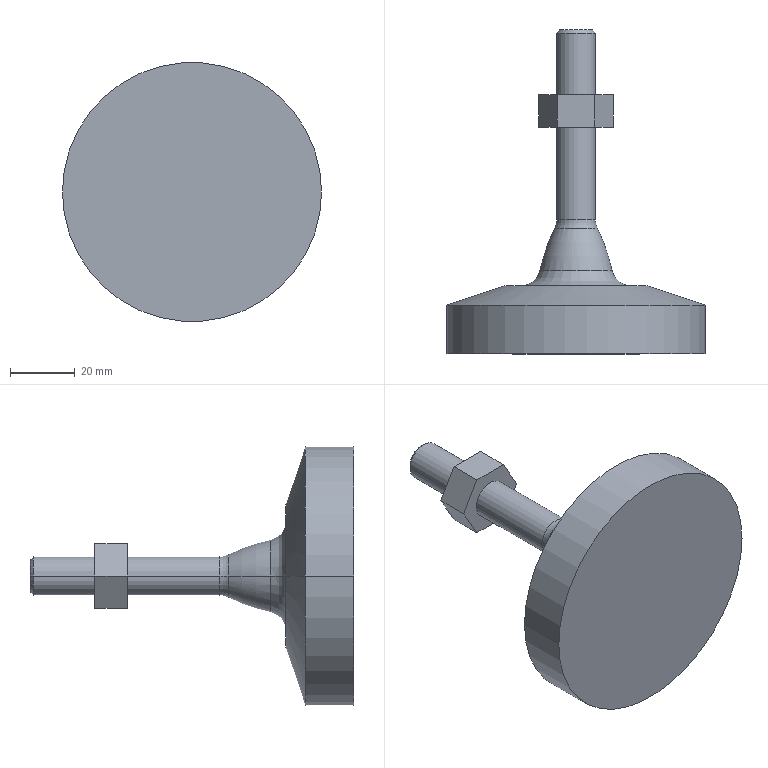Component | SolidWorks | FrameAssembly-1_FootCup-3 | 1 solid | 27 faces | box 80 x 100 x 80 mm | volume 109185 mm3 | plane 11 | torus 6 | cylinder 6 | cone 4 | commonest cylinder face diameters 12 x4 80 x2
build123d program:
from build123d import *

# Parameters (mm, degrees)
BOSS_EXTRUDE1_DEPTH = 10
FILLET1_R           = 6


with BuildPart() as part:
    # Sketch1 → Boss-Extrude1 (new body)
    with BuildSketch(Plane(origin=(0, 80, 0), x_dir=(1, 0, 0), z_dir=(0, 1, 0))):
        Polygon((-5.774, 10), (-11.547, 0), (-5.774, -10), (5.774, -10), (11.547, 0), (5.774, 10), align=None)
    extrude(amount=-BOSS_EXTRUDE1_DEPTH)

    # Sketch2 → Revolve1 (revolve)
    with BuildSketch(Plane(origin=(0, 0, 0), x_dir=(-1, 0, 0), z_dir=(0, 0, -1)), mode=Mode.PRIVATE) as revolve1_sk:
        with BuildLine():
            Line((-40, 0), (0, 0))
            Line((0, 0), (0, 70))
            Line((0, 70), (-6, 70))
            Line((-6, 70), (-6, 40))
            ThreePointArc((-6, 40), (-9.794, 30.751), (-12, 21))
            Line((-12, 21), (-22, 21))
            Line((-22, 21), (-40, 15))
            Line((-40, 15), (-40, 0))
        make_face()
    revolve(revolve1_sk.sketch.rotate(Axis((0, 0, 0), (0, 1, 0)), 180), axis=Axis((0, 0, 0), (0, 1, 0)))

    # Sketch3 → Revolve2 (revolve)
    with BuildSketch(Plane(origin=(0, 0, 0), x_dir=(-1, 0, 0), z_dir=(0, 0, -1)), mode=Mode.PRIVATE) as revolve2_sk:
        Polygon((-6, 80), (0, 80), (0, 100), (-5, 100), (-6, 99), align=None)
    revolve(revolve2_sk.sketch.rotate(Axis((0, 80, 0), (0, 1, 0)), 180), axis=Axis((0, 80, 0), (0, 1, 0)))

    # Fillet1
    fillet1_edges = [part.edges().sort_by_distance(p)[0] for p in [
        (6, 40, 0),
        (12, 21, 0),
    ]]
    fillet(fillet1_edges, radius=FILLET1_R)


solid = part.part

# Placed as in the assembly
solid = solid.moved(Location((-641.246, -528.627, -346.5), (0, 0, 0)))
STEP:
#1=COLOUR_RGB('',0.7922,0.8196,0.9333);
#2=FILL_AREA_STYLE_COLOUR('',#1);
#3=FILL_AREA_STYLE('',(#2));
#4=SURFACE_STYLE_FILL_AREA(#3);
#5=SURFACE_SIDE_STYLE('',(#4));
#6=SURFACE_STYLE_USAGE(.BOTH.,#5);
#7=PRESENTATION_STYLE_ASSIGNMENT((#6));
#8=CARTESIAN_POINT('',(-25.01,-19.182,-13.642));
#9=VERTEX_POINT('',#8);
#10=CARTESIAN_POINT('',(-25.482,-19.182,-13.642));
#11=VERTEX_POINT('',#10);
#12=CARTESIAN_POINT('',(-25.246,-19.182,-13.642));
#13=DIRECTION('',(0.,1.,0.));
#14=DIRECTION('',(-1.,0.,0.));
#15=AXIS2_PLACEMENT_3D('',#12,#13,#14);
#16=CIRCLE('',#15,0.2362);
#17=EDGE_CURVE('',#9,#11,#16,.T.);
#18=ORIENTED_EDGE('',*,*,#17,.F.);
#19=CARTESIAN_POINT('',(-24.986,-19.285,-13.642));
#20=VERTEX_POINT('',#19);
#21=CARTESIAN_POINT('',(-24.773,-19.182,-13.642));
#22=DIRECTION('',(-0.,0.,1.));
#23=DIRECTION('',(1.,0.,0.));
#24=AXIS2_PLACEMENT_3D('',#21,#22,#23);
#25=CIRCLE('',#24,0.2362);
#26=EDGE_CURVE('',#9,#20,#25,.T.);
#27=ORIENTED_EDGE('',*,*,#26,.T.);
#28=CARTESIAN_POINT('',(-25.506,-19.285,-13.642));
#29=VERTEX_POINT('',#28);
#30=CARTESIAN_POINT('',(-25.246,-19.285,-13.642));
#31=DIRECTION('',(-0.,-1.,0.));
#32=DIRECTION('',(1.,0.,0.));
#33=AXIS2_PLACEMENT_3D('',#30,#31,#32);
#34=CIRCLE('',#33,0.2598);
#35=EDGE_CURVE('',#29,#20,#34,.T.);
#36=ORIENTED_EDGE('',*,*,#35,.F.);
#37=CARTESIAN_POINT('',(-25.718,-19.182,-13.642));
#38=DIRECTION('',(0.,0.,-1.));
#39=DIRECTION('',(-1.,0.,0.));
#40=AXIS2_PLACEMENT_3D('',#37,#38,#39);
#41=CIRCLE('',#40,0.2362);
#42=EDGE_CURVE('',#11,#29,#41,.T.);
#43=ORIENTED_EDGE('',*,*,#42,.F.);
#44=EDGE_LOOP('',(#18,#27,#36,#43));
#45=FACE_OUTER_BOUND('',#44,.T.);
#46=CARTESIAN_POINT('',(-25.246,-19.182,-13.642));
#47=DIRECTION('',(0.,1.,0.));
#48=DIRECTION('',(-1.,0.,0.));
#49=AXIS2_PLACEMENT_3D('',#46,#47,#48);
#50=TOROIDAL_SURFACE('',#49,0.4724,0.2362);
#51=ADVANCED_FACE('',(#45),#50,.F.);
#52=CARTESIAN_POINT('',(-24.807,-19.8,-13.642));
#53=VERTEX_POINT('',#52);
#54=CARTESIAN_POINT('',(-25.685,-19.8,-13.642));
#55=VERTEX_POINT('',#54);
#56=CARTESIAN_POINT('',(-25.246,-19.8,-13.642));
#57=DIRECTION('',(0.,1.,0.));
#58=DIRECTION('',(1.,0.,0.));
#59=AXIS2_PLACEMENT_3D('',#56,#57,#58);
#60=CIRCLE('',#59,0.439);
#61=EDGE_CURVE('',#53,#55,#60,.T.);
#62=ORIENTED_EDGE('',*,*,#61,.F.);
#63=CARTESIAN_POINT('',(-24.576,-19.985,-13.642));
#64=VERTEX_POINT('',#63);
#65=CARTESIAN_POINT('',(-24.576,-19.749,-13.642));
#66=DIRECTION('',(-0.,0.,1.));
#67=DIRECTION('',(1.,0.,0.));
#68=AXIS2_PLACEMENT_3D('',#65,#66,#67);
#69=CIRCLE('',#68,0.2362);
#70=EDGE_CURVE('',#53,#64,#69,.T.);
#71=ORIENTED_EDGE('',*,*,#70,.T.);
#72=CARTESIAN_POINT('',(-25.916,-19.985,-13.642));
#73=VERTEX_POINT('',#72);
#74=CARTESIAN_POINT('',(-25.246,-19.985,-13.642));
#75=DIRECTION('',(-0.,-1.,0.));
#76=DIRECTION('',(-1.,0.,0.));
#77=AXIS2_PLACEMENT_3D('',#74,#75,#76);
#78=CIRCLE('',#77,0.6696);
#79=EDGE_CURVE('',#73,#64,#78,.T.);
#80=ORIENTED_EDGE('',*,*,#79,.F.);
#81=CARTESIAN_POINT('',(-25.916,-19.749,-13.642));
#82=DIRECTION('',(0.,0.,-1.));
#83=DIRECTION('',(-1.,0.,0.));
#84=AXIS2_PLACEMENT_3D('',#81,#82,#83);
#85=CIRCLE('',#84,0.2362);
#86=EDGE_CURVE('',#55,#73,#85,.T.);
#87=ORIENTED_EDGE('',*,*,#86,.F.);
#88=EDGE_LOOP('',(#62,#71,#80,#87));
#89=FACE_OUTER_BOUND('',#88,.T.);
#90=CARTESIAN_POINT('',(-25.246,-19.749,-13.642));
#91=DIRECTION('',(0.,1.,0.));
#92=DIRECTION('',(-1.,0.,0.));
#93=AXIS2_PLACEMENT_3D('',#90,#91,#92);
#94=TOROIDAL_SURFACE('',#93,0.6696,0.2362);
#95=ADVANCED_FACE('',(#89),#94,.F.);
#96=CARTESIAN_POINT('',(-25.443,-16.875,-13.642));
#97=VERTEX_POINT('',#96);
#98=CARTESIAN_POINT('',(-25.049,-16.875,-13.642));
#99=VERTEX_POINT('',#98);
#100=CARTESIAN_POINT('',(-25.246,-16.875,-13.642));
#101=DIRECTION('',(0.,1.,0.));
#102=DIRECTION('',(-1.,0.,0.));
#103=AXIS2_PLACEMENT_3D('',#100,#101,#102);
#104=CIRCLE('',#103,0.1969);
#105=EDGE_CURVE('',#97,#99,#104,.T.);
#106=ORIENTED_EDGE('',*,*,#105,.F.);
#107=CARTESIAN_POINT('',(-25.482,-16.914,-13.642));
#108=VERTEX_POINT('',#107);
#109=CARTESIAN_POINT('',(-25.443,-16.875,-13.642));
#110=DIRECTION('',(-0.7071,-0.7071,0.));
#111=VECTOR('',#110,39.37);
#112=LINE('',#109,#111);
#113=EDGE_CURVE('',#97,#108,#112,.T.);
#114=ORIENTED_EDGE('',*,*,#113,.T.);
#115=CARTESIAN_POINT('',(-25.01,-16.914,-13.642));
#116=VERTEX_POINT('',#115);
#117=CARTESIAN_POINT('',(-25.246,-16.914,-13.642));
#118=DIRECTION('',(0.,1.,0.));
#119=DIRECTION('',(-1.,0.,0.));
#120=AXIS2_PLACEMENT_3D('',#117,#118,#119);
#121=CIRCLE('',#120,0.2362);
#122=EDGE_CURVE('',#108,#116,#121,.T.);
#123=ORIENTED_EDGE('',*,*,#122,.T.);
#124=CARTESIAN_POINT('',(-25.049,-16.875,-13.642));
#125=DIRECTION('',(0.7071,-0.7071,0.));
#126=VECTOR('',#125,39.37);
#127=LINE('',#124,#126);
#128=EDGE_CURVE('',#99,#116,#127,.T.);
#129=ORIENTED_EDGE('',*,*,#128,.F.);
#130=EDGE_LOOP('',(#106,#114,#123,#129));
#131=FACE_OUTER_BOUND('',#130,.T.);
#132=CARTESIAN_POINT('',(-25.246,-16.875,-13.642));
#133=DIRECTION('',(-0.,-1.,0.));
#134=DIRECTION('',(1.,0.,0.));
#135=AXIS2_PLACEMENT_3D('',#132,#133,#134);
#136=CONICAL_SURFACE('',#135,0.1969,0.7854);
#137=ADVANCED_FACE('',(#131),#136,.T.);
#138=CARTESIAN_POINT('',(-25.482,-17.662,-13.642));
#139=VERTEX_POINT('',#138);
#140=CARTESIAN_POINT('',(-25.01,-17.662,-13.642));
#141=VERTEX_POINT('',#140);
#142=CARTESIAN_POINT('',(-25.246,-17.662,-13.642));
#143=DIRECTION('',(0.,1.,0.));
#144=DIRECTION('',(-1.,0.,0.));
#145=AXIS2_PLACEMENT_3D('',#142,#143,#144);
#146=CIRCLE('',#145,0.2362);
#147=EDGE_CURVE('',#139,#141,#146,.T.);
#148=ORIENTED_EDGE('',*,*,#147,.T.);
#149=CARTESIAN_POINT('',(-25.01,-17.662,-13.642));
#150=DIRECTION('',(0.,1.,0.));
#151=VECTOR('',#150,39.37);
#152=LINE('',#149,#151);
#153=EDGE_CURVE('',#141,#116,#152,.T.);
#154=ORIENTED_EDGE('',*,*,#153,.T.);
#155=ORIENTED_EDGE('',*,*,#122,.F.);
#156=CARTESIAN_POINT('',(-25.482,-17.662,-13.642));
#157=DIRECTION('',(0.,1.,0.));
#158=VECTOR('',#157,39.37);
#159=LINE('',#156,#158);
#160=EDGE_CURVE('',#139,#108,#159,.T.);
#161=ORIENTED_EDGE('',*,*,#160,.F.);
#162=EDGE_LOOP('',(#148,#154,#155,#161));
#163=FACE_OUTER_BOUND('',#162,.T.);
#164=CARTESIAN_POINT('',(-25.246,-17.662,-13.642));
#165=DIRECTION('',(0.,1.,0.));
#166=DIRECTION('',(-1.,0.,0.));
#167=AXIS2_PLACEMENT_3D('',#164,#165,#166);
#168=CYLINDRICAL_SURFACE('',#167,0.2362);
#169=ADVANCED_FACE('',(#163),#168,.T.);
#170=CARTESIAN_POINT('',(-26.112,-19.985,-13.642));
#171=VERTEX_POINT('',#170);
#172=CARTESIAN_POINT('',(-24.38,-19.985,-13.642));
#173=VERTEX_POINT('',#172);
#174=CARTESIAN_POINT('',(-25.246,-19.985,-13.642));
#175=DIRECTION('',(0.,1.,0.));
#176=DIRECTION('',(-1.,0.,0.));
#177=AXIS2_PLACEMENT_3D('',#174,#175,#176);
#178=CIRCLE('',#177,0.8661);
#179=EDGE_CURVE('',#171,#173,#178,.T.);
#180=ORIENTED_EDGE('',*,*,#179,.F.);
#181=CARTESIAN_POINT('',(-26.821,-20.222,-13.642));
#182=VERTEX_POINT('',#181);
#183=CARTESIAN_POINT('',(-26.112,-19.985,-13.642));
#184=DIRECTION('',(-0.9487,-0.3162,0.));
#185=VECTOR('',#184,39.37);
#186=LINE('',#183,#185);
#187=EDGE_CURVE('',#171,#182,#186,.T.);
#188=ORIENTED_EDGE('',*,*,#187,.T.);
#189=CARTESIAN_POINT('',(-23.671,-20.222,-13.642));
#190=VERTEX_POINT('',#189);
#191=CARTESIAN_POINT('',(-25.246,-20.222,-13.642));
#192=DIRECTION('',(0.,1.,0.));
#193=DIRECTION('',(-1.,0.,0.));
#194=AXIS2_PLACEMENT_3D('',#191,#192,#193);
#195=CIRCLE('',#194,1.575);
#196=EDGE_CURVE('',#182,#190,#195,.T.);
#197=ORIENTED_EDGE('',*,*,#196,.T.);
#198=CARTESIAN_POINT('',(-24.38,-19.985,-13.642));
#199=DIRECTION('',(0.9487,-0.3162,0.));
#200=VECTOR('',#199,39.37);
#201=LINE('',#198,#200);
#202=EDGE_CURVE('',#173,#190,#201,.T.);
#203=ORIENTED_EDGE('',*,*,#202,.F.);
#204=EDGE_LOOP('',(#180,#188,#197,#203));
#205=FACE_OUTER_BOUND('',#204,.T.);
#206=CARTESIAN_POINT('',(-25.246,-19.985,-13.642));
#207=DIRECTION('',(-0.,-1.,0.));
#208=DIRECTION('',(1.,0.,0.));
#209=AXIS2_PLACEMENT_3D('',#206,#207,#208);
#210=CONICAL_SURFACE('',#209,0.8661,1.249);
#211=ADVANCED_FACE('',(#205),#210,.T.);
#212=CARTESIAN_POINT('',(-25.246,-19.8,-13.642));
#213=DIRECTION('',(0.,1.,0.));
#214=DIRECTION('',(1.,0.,-0.));
#215=AXIS2_PLACEMENT_3D('',#212,#213,#214);
#216=CIRCLE('',#215,0.439);
#217=EDGE_CURVE('',#55,#53,#216,.T.);
#218=ORIENTED_EDGE('',*,*,#217,.T.);
#219=CARTESIAN_POINT('',(-27.113,-20.313,-13.642));
#220=DIRECTION('',(-0.,0.,1.));
#221=DIRECTION('',(1.,0.,0.));
#222=AXIS2_PLACEMENT_3D('',#219,#220,#221);
#223=CIRCLE('',#222,2.362);
#224=EDGE_CURVE('',#53,#20,#223,.T.);
#225=ORIENTED_EDGE('',*,*,#224,.T.);
#226=CARTESIAN_POINT('',(-25.246,-19.285,-13.642));
#227=DIRECTION('',(-0.,-1.,0.));
#228=DIRECTION('',(1.,0.,0.));
#229=AXIS2_PLACEMENT_3D('',#226,#227,#228);
#230=CIRCLE('',#229,0.2598);
#231=EDGE_CURVE('',#20,#29,#230,.T.);
#232=ORIENTED_EDGE('',*,*,#231,.T.);
#233=CARTESIAN_POINT('',(-23.379,-20.313,-13.642));
#234=DIRECTION('',(0.,0.,-1.));
#235=DIRECTION('',(-1.,0.,0.));
#236=AXIS2_PLACEMENT_3D('',#233,#234,#235);
#237=CIRCLE('',#236,2.362);
#238=EDGE_CURVE('',#55,#29,#237,.T.);
#239=ORIENTED_EDGE('',*,*,#238,.F.);
#240=EDGE_LOOP('',(#218,#225,#232,#239));
#241=FACE_OUTER_BOUND('',#240,.T.);
#242=CARTESIAN_POINT('',(-25.246,-20.313,-13.642));
#243=DIRECTION('',(0.,1.,0.));
#244=DIRECTION('',(-1.,0.,0.));
#245=AXIS2_PLACEMENT_3D('',#242,#243,#244);
#246=TOROIDAL_SURFACE('',#245,-1.867,2.362);
#247=ADVANCED_FACE('',(#241),#246,.T.);
#248=CARTESIAN_POINT('',(-25.246,-19.182,-13.642));
#249=DIRECTION('',(0.,1.,0.));
#250=DIRECTION('',(-1.,0.,0.));
#251=AXIS2_PLACEMENT_3D('',#248,#249,#250);
#252=CIRCLE('',#251,0.2362);
#253=EDGE_CURVE('',#11,#9,#252,.T.);
#254=ORIENTED_EDGE('',*,*,#253,.T.);
#255=CARTESIAN_POINT('',(-25.01,-18.056,-13.642));
#256=VERTEX_POINT('',#255);
#257=CARTESIAN_POINT('',(-25.01,-20.812,-13.642));
#258=DIRECTION('',(0.,1.,0.));
#259=VECTOR('',#258,39.37);
#260=LINE('',#257,#259);
#261=EDGE_CURVE('',#9,#256,#260,.T.);
#262=ORIENTED_EDGE('',*,*,#261,.T.);
#263=CARTESIAN_POINT('',(-25.482,-18.056,-13.642));
#264=VERTEX_POINT('',#263);
#265=CARTESIAN_POINT('',(-25.246,-18.056,-13.642));
#266=DIRECTION('',(0.,1.,0.));
#267=DIRECTION('',(-1.,0.,0.));
#268=AXIS2_PLACEMENT_3D('',#265,#266,#267);
#269=CIRCLE('',#268,0.2362);
#270=EDGE_CURVE('',#264,#256,#269,.T.);
#271=ORIENTED_EDGE('',*,*,#270,.F.);
#272=CARTESIAN_POINT('',(-25.482,-20.812,-13.642));
#273=DIRECTION('',(0.,1.,0.));
#274=VECTOR('',#273,39.37);
#275=LINE('',#272,#274);
#276=EDGE_CURVE('',#11,#264,#275,.T.);
#277=ORIENTED_EDGE('',*,*,#276,.F.);
#278=EDGE_LOOP('',(#254,#262,#271,#277));
#279=FACE_OUTER_BOUND('',#278,.T.);
#280=CARTESIAN_POINT('',(-25.246,-20.812,-13.642));
#281=DIRECTION('',(0.,1.,0.));
#282=DIRECTION('',(-1.,0.,0.));
#283=AXIS2_PLACEMENT_3D('',#280,#281,#282);
#284=CYLINDRICAL_SURFACE('',#283,0.2362);
#285=ADVANCED_FACE('',(#279),#284,.T.);
#286=CARTESIAN_POINT('',(-26.821,-20.812,-13.642));
#287=VERTEX_POINT('',#286);
#288=CARTESIAN_POINT('',(-23.671,-20.812,-13.642));
#289=VERTEX_POINT('',#288);
#290=CARTESIAN_POINT('',(-25.246,-20.812,-13.642));
#291=DIRECTION('',(0.,1.,0.));
#292=DIRECTION('',(-1.,0.,0.));
#293=AXIS2_PLACEMENT_3D('',#290,#291,#292);
#294=CIRCLE('',#293,1.575);
#295=EDGE_CURVE('',#287,#289,#294,.T.);
#296=ORIENTED_EDGE('',*,*,#295,.T.);
#297=CARTESIAN_POINT('',(-23.671,-20.812,-13.642));
#298=DIRECTION('',(0.,1.,0.));
#299=VECTOR('',#298,39.37);
#300=LINE('',#297,#299);
#301=EDGE_CURVE('',#289,#190,#300,.T.);
#302=ORIENTED_EDGE('',*,*,#301,.T.);
#303=ORIENTED_EDGE('',*,*,#196,.F.);
#304=CARTESIAN_POINT('',(-26.821,-20.812,-13.642));
#305=DIRECTION('',(0.,1.,0.));
#306=VECTOR('',#305,39.37);
#307=LINE('',#304,#306);
#308=EDGE_CURVE('',#287,#182,#307,.T.);
#309=ORIENTED_EDGE('',*,*,#308,.F.);
#310=EDGE_LOOP('',(#296,#302,#303,#309));
#311=FACE_OUTER_BOUND('',#310,.T.);
#312=CARTESIAN_POINT('',(-25.246,-20.812,-13.642));
#313=DIRECTION('',(0.,1.,0.));
#314=DIRECTION('',(-1.,0.,0.));
#315=AXIS2_PLACEMENT_3D('',#312,#313,#314);
#316=CYLINDRICAL_SURFACE('',#315,1.575);
#317=ADVANCED_FACE('',(#311),#316,.T.);
#318=CARTESIAN_POINT('',(-25.019,-17.662,-14.035));
#319=VERTEX_POINT('',#318);
#320=CARTESIAN_POINT('',(-25.473,-17.662,-14.035));
#321=VERTEX_POINT('',#320);
#322=CARTESIAN_POINT('',(-25.019,-17.662,-14.035));
#323=DIRECTION('',(-1.,0.,0.));
#324=VECTOR('',#323,39.37);
#325=LINE('',#322,#324);
#326=EDGE_CURVE('',#319,#321,#325,.T.);
#327=ORIENTED_EDGE('',*,*,#326,.F.);
#328=CARTESIAN_POINT('',(-25.019,-18.056,-14.035));
#329=VERTEX_POINT('',#328);
#330=CARTESIAN_POINT('',(-25.019,-18.056,-14.035));
#331=DIRECTION('',(0.,1.,0.));
#332=VECTOR('',#331,39.37);
#333=LINE('',#330,#332);
#334=EDGE_CURVE('',#329,#319,#333,.T.);
#335=ORIENTED_EDGE('',*,*,#334,.F.);
#336=CARTESIAN_POINT('',(-25.473,-18.056,-14.035));
#337=VERTEX_POINT('',#336);
#338=CARTESIAN_POINT('',(-25.019,-18.056,-14.035));
#339=DIRECTION('',(-1.,0.,0.));
#340=VECTOR('',#339,39.37);
#341=LINE('',#338,#340);
#342=EDGE_CURVE('',#329,#337,#341,.T.);
#343=ORIENTED_EDGE('',*,*,#342,.T.);
#344=CARTESIAN_POINT('',(-25.473,-18.056,-14.035));
#345=DIRECTION('',(0.,1.,0.));
#346=VECTOR('',#345,39.37);
#347=LINE('',#344,#346);
#348=EDGE_CURVE('',#337,#321,#347,.T.);
#349=ORIENTED_EDGE('',*,*,#348,.T.);
#350=EDGE_LOOP('',(#327,#335,#343,#349));
#351=FACE_OUTER_BOUND('',#350,.T.);
#352=CARTESIAN_POINT('',(-25.019,-18.056,-14.035));
#353=DIRECTION('',(-0.,0.,-1.));
#354=DIRECTION('',(-1.,0.,0.));
#355=AXIS2_PLACEMENT_3D('',#352,#353,#354);
#356=PLANE('',#355);
#357=ADVANCED_FACE('',(#351),#356,.T.);
#358=CARTESIAN_POINT('',(-24.791,-17.662,-13.642));
#359=VERTEX_POINT('',#358);
#360=CARTESIAN_POINT('',(-24.791,-17.662,-13.642));
#361=DIRECTION('',(-0.5,0.,-0.866));
#362=VECTOR('',#361,39.37);
#363=LINE('',#360,#362);
#364=EDGE_CURVE('',#359,#319,#363,.T.);
#365=ORIENTED_EDGE('',*,*,#364,.F.);
#366=CARTESIAN_POINT('',(-24.791,-18.056,-13.642));
#367=VERTEX_POINT('',#366);
#368=CARTESIAN_POINT('',(-24.791,-18.056,-13.642));
#369=DIRECTION('',(0.,1.,0.));
#370=VECTOR('',#369,39.37);
#371=LINE('',#368,#370);
#372=EDGE_CURVE('',#367,#359,#371,.T.);
#373=ORIENTED_EDGE('',*,*,#372,.F.);
#374=CARTESIAN_POINT('',(-24.791,-18.056,-13.642));
#375=DIRECTION('',(-0.5,0.,-0.866));
#376=VECTOR('',#375,39.37);
#377=LINE('',#374,#376);
#378=EDGE_CURVE('',#367,#329,#377,.T.);
#379=ORIENTED_EDGE('',*,*,#378,.T.);
#380=ORIENTED_EDGE('',*,*,#334,.T.);
#381=EDGE_LOOP('',(#365,#373,#379,#380));
#382=FACE_OUTER_BOUND('',#381,.T.);
#383=CARTESIAN_POINT('',(-24.791,-18.056,-13.642));
#384=DIRECTION('',(0.866,0.,-0.5));
#385=DIRECTION('',(-0.5,0.,-0.866));
#386=AXIS2_PLACEMENT_3D('',#383,#384,#385);
#387=PLANE('',#386);
#388=ADVANCED_FACE('',(#382),#387,.T.);
#389=CARTESIAN_POINT('',(-25.019,-17.662,-13.248));
#390=VERTEX_POINT('',#389);
#391=CARTESIAN_POINT('',(-25.019,-17.662,-13.248));
#392=DIRECTION('',(0.5,0.,-0.866));
#393=VECTOR('',#392,39.37);
#394=LINE('',#391,#393);
#395=EDGE_CURVE('',#390,#359,#394,.T.);
#396=ORIENTED_EDGE('',*,*,#395,.F.);
#397=CARTESIAN_POINT('',(-25.019,-18.056,-13.248));
#398=VERTEX_POINT('',#397);
#399=CARTESIAN_POINT('',(-25.019,-18.056,-13.248));
#400=DIRECTION('',(0.,1.,0.));
#401=VECTOR('',#400,39.37);
#402=LINE('',#399,#401);
#403=EDGE_CURVE('',#398,#390,#402,.T.);
#404=ORIENTED_EDGE('',*,*,#403,.F.);
#405=CARTESIAN_POINT('',(-25.019,-18.056,-13.248));
#406=DIRECTION('',(0.5,0.,-0.866));
#407=VECTOR('',#406,39.37);
#408=LINE('',#405,#407);
#409=EDGE_CURVE('',#398,#367,#408,.T.);
#410=ORIENTED_EDGE('',*,*,#409,.T.);
#411=ORIENTED_EDGE('',*,*,#372,.T.);
#412=EDGE_LOOP('',(#396,#404,#410,#411));
#413=FACE_OUTER_BOUND('',#412,.T.);
#414=CARTESIAN_POINT('',(-25.019,-18.056,-13.248));
#415=DIRECTION('',(0.866,0.,0.5));
#416=DIRECTION('',(0.5,0.,-0.866));
#417=AXIS2_PLACEMENT_3D('',#414,#415,#416);
#418=PLANE('',#417);
#419=ADVANCED_FACE('',(#413),#418,.T.);
#420=CARTESIAN_POINT('',(-25.473,-17.662,-13.248));
#421=VERTEX_POINT('',#420);
#422=CARTESIAN_POINT('',(-25.473,-17.662,-13.248));
#423=DIRECTION('',(1.,0.,0.));
#424=VECTOR('',#423,39.37);
#425=LINE('',#422,#424);
#426=EDGE_CURVE('',#421,#390,#425,.T.);
#427=ORIENTED_EDGE('',*,*,#426,.F.);
#428=CARTESIAN_POINT('',(-25.473,-18.056,-13.248));
#429=VERTEX_POINT('',#428);
#430=CARTESIAN_POINT('',(-25.473,-18.056,-13.248));
#431=DIRECTION('',(0.,1.,0.));
#432=VECTOR('',#431,39.37);
#433=LINE('',#430,#432);
#434=EDGE_CURVE('',#429,#421,#433,.T.);
#435=ORIENTED_EDGE('',*,*,#434,.F.);
#436=CARTESIAN_POINT('',(-25.473,-18.056,-13.248));
#437=DIRECTION('',(1.,0.,0.));
#438=VECTOR('',#437,39.37);
#439=LINE('',#436,#438);
#440=EDGE_CURVE('',#429,#398,#439,.T.);
#441=ORIENTED_EDGE('',*,*,#440,.T.);
#442=ORIENTED_EDGE('',*,*,#403,.T.);
#443=EDGE_LOOP('',(#427,#435,#441,#442));
#444=FACE_OUTER_BOUND('',#443,.T.);
#445=CARTESIAN_POINT('',(-25.473,-18.056,-13.248));
#446=DIRECTION('',(0.,0.,1.));
#447=DIRECTION('',(1.,0.,0.));
#448=AXIS2_PLACEMENT_3D('',#445,#446,#447);
#449=PLANE('',#448);
#450=ADVANCED_FACE('',(#444),#449,.T.);
#451=CARTESIAN_POINT('',(-25.701,-17.662,-13.642));
#452=VERTEX_POINT('',#451);
#453=CARTESIAN_POINT('',(-25.701,-17.662,-13.642));
#454=DIRECTION('',(0.5,0.,0.866));
#455=VECTOR('',#454,39.37);
#456=LINE('',#453,#455);
#457=EDGE_CURVE('',#452,#421,#456,.T.);
#458=ORIENTED_EDGE('',*,*,#457,.F.);
#459=CARTESIAN_POINT('',(-25.701,-18.056,-13.642));
#460=VERTEX_POINT('',#459);
#461=CARTESIAN_POINT('',(-25.701,-18.056,-13.642));
#462=DIRECTION('',(0.,1.,0.));
#463=VECTOR('',#462,39.37);
#464=LINE('',#461,#463);
#465=EDGE_CURVE('',#460,#452,#464,.T.);
#466=ORIENTED_EDGE('',*,*,#465,.F.);
#467=CARTESIAN_POINT('',(-25.701,-18.056,-13.642));
#468=DIRECTION('',(0.5,0.,0.866));
#469=VECTOR('',#468,39.37);
#470=LINE('',#467,#469);
#471=EDGE_CURVE('',#460,#429,#470,.T.);
#472=ORIENTED_EDGE('',*,*,#471,.T.);
#473=ORIENTED_EDGE('',*,*,#434,.T.);
#474=EDGE_LOOP('',(#458,#466,#472,#473));
#475=FACE_OUTER_BOUND('',#474,.T.);
#476=CARTESIAN_POINT('',(-25.701,-18.056,-13.642));
#477=DIRECTION('',(-0.866,0.,0.5));
#478=DIRECTION('',(0.5,0.,0.866));
#479=AXIS2_PLACEMENT_3D('',#476,#477,#478);
#480=PLANE('',#479);
#481=ADVANCED_FACE('',(#475),#480,.T.);
#482=CARTESIAN_POINT('',(-25.473,-17.662,-14.035));
#483=DIRECTION('',(-0.5,0.,0.866));
#484=VECTOR('',#483,39.37);
#485=LINE('',#482,#484);
#486=EDGE_CURVE('',#321,#452,#485,.T.);
#487=ORIENTED_EDGE('',*,*,#486,.F.);
#488=ORIENTED_EDGE('',*,*,#348,.F.);
#489=CARTESIAN_POINT('',(-25.473,-18.056,-14.035));
#490=DIRECTION('',(-0.5,0.,0.866));
#491=VECTOR('',#490,39.37);
#492=LINE('',#489,#491);
#493=EDGE_CURVE('',#337,#460,#492,.T.);
#494=ORIENTED_EDGE('',*,*,#493,.T.);
#495=ORIENTED_EDGE('',*,*,#465,.T.);
#496=EDGE_LOOP('',(#487,#488,#494,#495));
#497=FACE_OUTER_BOUND('',#496,.T.);
#498=CARTESIAN_POINT('',(-25.473,-18.056,-14.035));
#499=DIRECTION('',(-0.866,0.,-0.5));
#500=DIRECTION('',(-0.5,0.,0.866));
#501=AXIS2_PLACEMENT_3D('',#498,#499,#500);
#502=PLANE('',#501);
#503=ADVANCED_FACE('',(#497),#502,.T.);
#504=ORIENTED_EDGE('',*,*,#270,.T.);
#505=CARTESIAN_POINT('',(-25.246,-18.056,-13.642));
#506=DIRECTION('',(0.,1.,0.));
#507=DIRECTION('',(-1.,0.,0.));
#508=AXIS2_PLACEMENT_3D('',#505,#506,#507);
#509=CIRCLE('',#508,0.2362);
#510=EDGE_CURVE('',#256,#264,#509,.T.);
#511=ORIENTED_EDGE('',*,*,#510,.T.);
#512=EDGE_LOOP('',(#504,#511));
#513=FACE_BOUND('',#512,.T.);
#514=ORIENTED_EDGE('',*,*,#342,.F.);
#515=ORIENTED_EDGE('',*,*,#378,.F.);
#516=ORIENTED_EDGE('',*,*,#409,.F.);
#517=ORIENTED_EDGE('',*,*,#440,.F.);
#518=ORIENTED_EDGE('',*,*,#471,.F.);
#519=ORIENTED_EDGE('',*,*,#493,.F.);
#520=EDGE_LOOP('',(#514,#515,#516,#517,#518,#519));
#521=FACE_OUTER_BOUND('',#520,.T.);
#522=CARTESIAN_POINT('',(-25.246,-18.056,-13.642));
#523=DIRECTION('',(0.,1.,0.));
#524=DIRECTION('',(0.,0.,1.));
#525=AXIS2_PLACEMENT_3D('',#522,#523,#524);
#526=PLANE('',#525);
#527=ADVANCED_FACE('',(#513,#521),#526,.F.);
#528=ORIENTED_EDGE('',*,*,#147,.F.);
#529=CARTESIAN_POINT('',(-25.246,-17.662,-13.642));
#530=DIRECTION('',(0.,1.,0.));
#531=DIRECTION('',(-1.,0.,0.));
#532=AXIS2_PLACEMENT_3D('',#529,#530,#531);
#533=CIRCLE('',#532,0.2362);
#534=EDGE_CURVE('',#141,#139,#533,.T.);
#535=ORIENTED_EDGE('',*,*,#534,.F.);
#536=EDGE_LOOP('',(#528,#535));
#537=FACE_BOUND('',#536,.T.);
#538=ORIENTED_EDGE('',*,*,#326,.T.);
#539=ORIENTED_EDGE('',*,*,#486,.T.);
#540=ORIENTED_EDGE('',*,*,#457,.T.);
#541=ORIENTED_EDGE('',*,*,#426,.T.);
#542=ORIENTED_EDGE('',*,*,#395,.T.);
#543=ORIENTED_EDGE('',*,*,#364,.T.);
#544=EDGE_LOOP('',(#538,#539,#540,#541,#542,#543));
#545=FACE_OUTER_BOUND('',#544,.T.);
#546=CARTESIAN_POINT('',(-25.246,-17.662,-13.642));
#547=DIRECTION('',(0.,1.,0.));
#548=DIRECTION('',(0.,0.,1.));
#549=AXIS2_PLACEMENT_3D('',#546,#547,#548);
#550=PLANE('',#549);
#551=ADVANCED_FACE('',(#537,#545),#550,.T.);
#552=ORIENTED_EDGE('',*,*,#301,.F.);
#553=CARTESIAN_POINT('',(-25.246,-20.812,-13.642));
#554=DIRECTION('',(0.,1.,0.));
#555=DIRECTION('',(-1.,0.,0.));
#556=AXIS2_PLACEMENT_3D('',#553,#554,#555);
#557=CIRCLE('',#556,1.575);
#558=EDGE_CURVE('',#289,#287,#557,.T.);
#559=ORIENTED_EDGE('',*,*,#558,.T.);
#560=ORIENTED_EDGE('',*,*,#308,.T.);
#561=CARTESIAN_POINT('',(-25.246,-20.222,-13.642));
#562=DIRECTION('',(0.,1.,0.));
#563=DIRECTION('',(-1.,0.,0.));
#564=AXIS2_PLACEMENT_3D('',#561,#562,#563);
#565=CIRCLE('',#564,1.575);
#566=EDGE_CURVE('',#190,#182,#565,.T.);
#567=ORIENTED_EDGE('',*,*,#566,.F.);
#568=EDGE_LOOP('',(#552,#559,#560,#567));
#569=FACE_OUTER_BOUND('',#568,.T.);
#570=CARTESIAN_POINT('',(-25.246,-20.812,-13.642));
#571=DIRECTION('',(0.,1.,0.));
#572=DIRECTION('',(-1.,0.,0.));
#573=AXIS2_PLACEMENT_3D('',#570,#571,#572);
#574=CYLINDRICAL_SURFACE('',#573,1.575);
#575=ADVANCED_FACE('',(#569),#574,.T.);
#576=ORIENTED_EDGE('',*,*,#295,.F.);
#577=ORIENTED_EDGE('',*,*,#558,.F.);
#578=EDGE_LOOP('',(#576,#577));
#579=FACE_OUTER_BOUND('',#578,.T.);
#580=CARTESIAN_POINT('',(-23.671,-20.812,-13.642));
#581=DIRECTION('',(-0.,-1.,0.));
#582=DIRECTION('',(1.,-0.,0.));
#583=AXIS2_PLACEMENT_3D('',#580,#581,#582);
#584=PLANE('',#583);
#585=ADVANCED_FACE('',(#579),#584,.T.);
#586=ORIENTED_EDGE('',*,*,#261,.F.);
#587=ORIENTED_EDGE('',*,*,#17,.T.);
#588=ORIENTED_EDGE('',*,*,#276,.T.);
#589=ORIENTED_EDGE('',*,*,#510,.F.);
#590=EDGE_LOOP('',(#586,#587,#588,#589));
#591=FACE_OUTER_BOUND('',#590,.T.);
#592=CARTESIAN_POINT('',(-25.246,-20.812,-13.642));
#593=DIRECTION('',(0.,1.,0.));
#594=DIRECTION('',(-1.,0.,0.));
#595=AXIS2_PLACEMENT_3D('',#592,#593,#594);
#596=CYLINDRICAL_SURFACE('',#595,0.2362);
#597=ADVANCED_FACE('',(#591),#596,.T.);
#598=ORIENTED_EDGE('',*,*,#224,.F.);
#599=ORIENTED_EDGE('',*,*,#61,.T.);
#600=ORIENTED_EDGE('',*,*,#238,.T.);
#601=ORIENTED_EDGE('',*,*,#35,.T.);
#602=EDGE_LOOP('',(#598,#599,#600,#601));
#603=FACE_OUTER_BOUND('',#602,.T.);
#604=CARTESIAN_POINT('',(-25.246,-20.313,-13.642));
#605=DIRECTION('',(0.,1.,0.));
#606=DIRECTION('',(-1.,0.,0.));
#607=AXIS2_PLACEMENT_3D('',#604,#605,#606);
#608=TOROIDAL_SURFACE('',#607,-1.867,2.362);
#609=ADVANCED_FACE('',(#603),#608,.T.);
#610=ORIENTED_EDGE('',*,*,#79,.T.);
#611=CARTESIAN_POINT('',(-25.246,-19.985,-13.642));
#612=DIRECTION('',(-0.,-1.,0.));
#613=DIRECTION('',(-1.,0.,0.));
#614=AXIS2_PLACEMENT_3D('',#611,#612,#613);
#615=CIRCLE('',#614,0.6696);
#616=EDGE_CURVE('',#64,#73,#615,.T.);
#617=ORIENTED_EDGE('',*,*,#616,.T.);
#618=EDGE_LOOP('',(#610,#617));
#619=FACE_BOUND('',#618,.T.);
#620=CARTESIAN_POINT('',(-25.246,-19.985,-13.642));
#621=DIRECTION('',(0.,1.,0.));
#622=DIRECTION('',(-1.,0.,0.));
#623=AXIS2_PLACEMENT_3D('',#620,#621,#622);
#624=CIRCLE('',#623,0.8661);
#625=EDGE_CURVE('',#173,#171,#624,.T.);
#626=ORIENTED_EDGE('',*,*,#625,.T.);
#627=ORIENTED_EDGE('',*,*,#179,.T.);
#628=EDGE_LOOP('',(#626,#627));
#629=FACE_OUTER_BOUND('',#628,.T.);
#630=CARTESIAN_POINT('',(-24.773,-19.985,-13.642));
#631=DIRECTION('',(0.,1.,0.));
#632=DIRECTION('',(-1.,0.,0.));
#633=AXIS2_PLACEMENT_3D('',#630,#631,#632);
#634=PLANE('',#633);
#635=ADVANCED_FACE('',(#619,#629),#634,.T.);
#636=ORIENTED_EDGE('',*,*,#187,.F.);
#637=ORIENTED_EDGE('',*,*,#625,.F.);
#638=ORIENTED_EDGE('',*,*,#202,.T.);
#639=ORIENTED_EDGE('',*,*,#566,.T.);
#640=EDGE_LOOP('',(#636,#637,#638,#639));
#641=FACE_OUTER_BOUND('',#640,.T.);
#642=CARTESIAN_POINT('',(-25.246,-19.985,-13.642));
#643=DIRECTION('',(-0.,-1.,0.));
#644=DIRECTION('',(1.,0.,0.));
#645=AXIS2_PLACEMENT_3D('',#642,#643,#644);
#646=CONICAL_SURFACE('',#645,0.8661,1.249);
#647=ADVANCED_FACE('',(#641),#646,.T.);
#648=ORIENTED_EDGE('',*,*,#153,.F.);
#649=ORIENTED_EDGE('',*,*,#534,.T.);
#650=ORIENTED_EDGE('',*,*,#160,.T.);
#651=CARTESIAN_POINT('',(-25.246,-16.914,-13.642));
#652=DIRECTION('',(0.,1.,0.));
#653=DIRECTION('',(-1.,0.,0.));
#654=AXIS2_PLACEMENT_3D('',#651,#652,#653);
#655=CIRCLE('',#654,0.2362);
#656=EDGE_CURVE('',#116,#108,#655,.T.);
#657=ORIENTED_EDGE('',*,*,#656,.F.);
#658=EDGE_LOOP('',(#648,#649,#650,#657));
#659=FACE_OUTER_BOUND('',#658,.T.);
#660=CARTESIAN_POINT('',(-25.246,-17.662,-13.642));
#661=DIRECTION('',(0.,1.,0.));
#662=DIRECTION('',(-1.,0.,0.));
#663=AXIS2_PLACEMENT_3D('',#660,#661,#662);
#664=CYLINDRICAL_SURFACE('',#663,0.2362);
#665=ADVANCED_FACE('',(#659),#664,.T.);
#666=CARTESIAN_POINT('',(-25.246,-16.875,-13.642));
#667=DIRECTION('',(0.,1.,0.));
#668=DIRECTION('',(-1.,0.,0.));
#669=AXIS2_PLACEMENT_3D('',#666,#667,#668);
#670=CIRCLE('',#669,0.1969);
#671=EDGE_CURVE('',#99,#97,#670,.T.);
#672=ORIENTED_EDGE('',*,*,#671,.T.);
#673=ORIENTED_EDGE('',*,*,#105,.T.);
#674=EDGE_LOOP('',(#672,#673));
#675=FACE_OUTER_BOUND('',#674,.T.);
#676=CARTESIAN_POINT('',(-25.246,-16.875,-13.642));
#677=DIRECTION('',(0.,1.,0.));
#678=DIRECTION('',(-1.,0.,0.));
#679=AXIS2_PLACEMENT_3D('',#676,#677,#678);
#680=PLANE('',#679);
#681=ADVANCED_FACE('',(#675),#680,.T.);
#682=ORIENTED_EDGE('',*,*,#113,.F.);
#683=ORIENTED_EDGE('',*,*,#671,.F.);
#684=ORIENTED_EDGE('',*,*,#128,.T.);
#685=ORIENTED_EDGE('',*,*,#656,.T.);
#686=EDGE_LOOP('',(#682,#683,#684,#685));
#687=FACE_OUTER_BOUND('',#686,.T.);
#688=CARTESIAN_POINT('',(-25.246,-16.875,-13.642));
#689=DIRECTION('',(-0.,-1.,0.));
#690=DIRECTION('',(1.,0.,0.));
#691=AXIS2_PLACEMENT_3D('',#688,#689,#690);
#692=CONICAL_SURFACE('',#691,0.1969,0.7854);
#693=ADVANCED_FACE('',(#687),#692,.T.);
#694=ORIENTED_EDGE('',*,*,#70,.F.);
#695=ORIENTED_EDGE('',*,*,#217,.F.);
#696=ORIENTED_EDGE('',*,*,#86,.T.);
#697=ORIENTED_EDGE('',*,*,#616,.F.);
#698=EDGE_LOOP('',(#694,#695,#696,#697));
#699=FACE_OUTER_BOUND('',#698,.T.);
#700=CARTESIAN_POINT('',(-25.246,-19.749,-13.642));
#701=DIRECTION('',(0.,1.,0.));
#702=DIRECTION('',(-1.,0.,0.));
#703=AXIS2_PLACEMENT_3D('',#700,#701,#702);
#704=TOROIDAL_SURFACE('',#703,0.6696,0.2362);
#705=ADVANCED_FACE('',(#699),#704,.F.);
#706=ORIENTED_EDGE('',*,*,#26,.F.);
#707=ORIENTED_EDGE('',*,*,#253,.F.);
#708=ORIENTED_EDGE('',*,*,#42,.T.);
#709=ORIENTED_EDGE('',*,*,#231,.F.);
#710=EDGE_LOOP('',(#706,#707,#708,#709));
#711=FACE_OUTER_BOUND('',#710,.T.);
#712=CARTESIAN_POINT('',(-25.246,-19.182,-13.642));
#713=DIRECTION('',(0.,1.,0.));
#714=DIRECTION('',(-1.,0.,0.));
#715=AXIS2_PLACEMENT_3D('',#712,#713,#714);
#716=TOROIDAL_SURFACE('',#715,0.4724,0.2362);
#717=ADVANCED_FACE('',(#711),#716,.F.);
#718=CLOSED_SHELL('',(#51,#95,#137,#169,#211,#247,#285,#317,#357,#388,#419,#450,#481,#503,#527,#551,#575,#585,#597,#609,#635,#647,#665,#681,#693,#705,#717));
#719=MANIFOLD_SOLID_BREP('',#718);
#720=STYLED_ITEM('',(#7),#719);
#721=PRESENTATION_LAYER_ASSIGNMENT('','',(#720));
#722=CARTESIAN_POINT('',(0.,0.,0.));
#723=DIRECTION('',(0.,0.,1.));
#724=DIRECTION('',(1.,0.,0.));
#725=AXIS2_PLACEMENT_3D('',#722,#723,#724);
#726=(LENGTH_UNIT()NAMED_UNIT(*)SI_UNIT($,.METRE.));
#727=LENGTH_MEASURE_WITH_UNIT(LENGTH_MEASURE(0.0254),#726);
#728=DIMENSIONAL_EXPONENTS(1.,0.,0.,0.,0.,0.,0.);
#729=(CONVERSION_BASED_UNIT('',#727)LENGTH_UNIT()NAMED_UNIT(#728));
#730=UNCERTAINTY_MEASURE_WITH_UNIT(LENGTH_MEASURE(0.00001),#729,'','');
#731=(NAMED_UNIT(*)PLANE_ANGLE_UNIT()SI_UNIT($,.RADIAN.));
#732=(NAMED_UNIT(*)SI_UNIT($,.STERADIAN.)SOLID_ANGLE_UNIT());
#733=(GEOMETRIC_REPRESENTATION_CONTEXT(3)GLOBAL_UNCERTAINTY_ASSIGNED_CONTEXT((#730))GLOBAL_UNIT_ASSIGNED_CONTEXT((#729,#731,#732))REPRESENTATION_CONTEXT('',''));
#734=ADVANCED_BREP_SHAPE_REPRESENTATION('',(#719,#725),#733);
#735=(LENGTH_UNIT()NAMED_UNIT(*)SI_UNIT($,.METRE.));
#736=LENGTH_MEASURE_WITH_UNIT(LENGTH_MEASURE(0.0254),#735);
#737=DIMENSIONAL_EXPONENTS(1.,0.,0.,0.,0.,0.,0.);
#738=(CONVERSION_BASED_UNIT('',#736)LENGTH_UNIT()NAMED_UNIT(#737));
#739=UNCERTAINTY_MEASURE_WITH_UNIT(LENGTH_MEASURE(0.00001),#738,'','');
#740=(NAMED_UNIT(*)PLANE_ANGLE_UNIT()SI_UNIT($,.RADIAN.));
#741=(NAMED_UNIT(*)SI_UNIT($,.STERADIAN.)SOLID_ANGLE_UNIT());
#742=(GEOMETRIC_REPRESENTATION_CONTEXT(3)GLOBAL_UNCERTAINTY_ASSIGNED_CONTEXT((#739))GLOBAL_UNIT_ASSIGNED_CONTEXT((#738,#740,#741))REPRESENTATION_CONTEXT('',''));
#743=MECHANICAL_DESIGN_GEOMETRIC_PRESENTATION_REPRESENTATION('',(#720),#742);